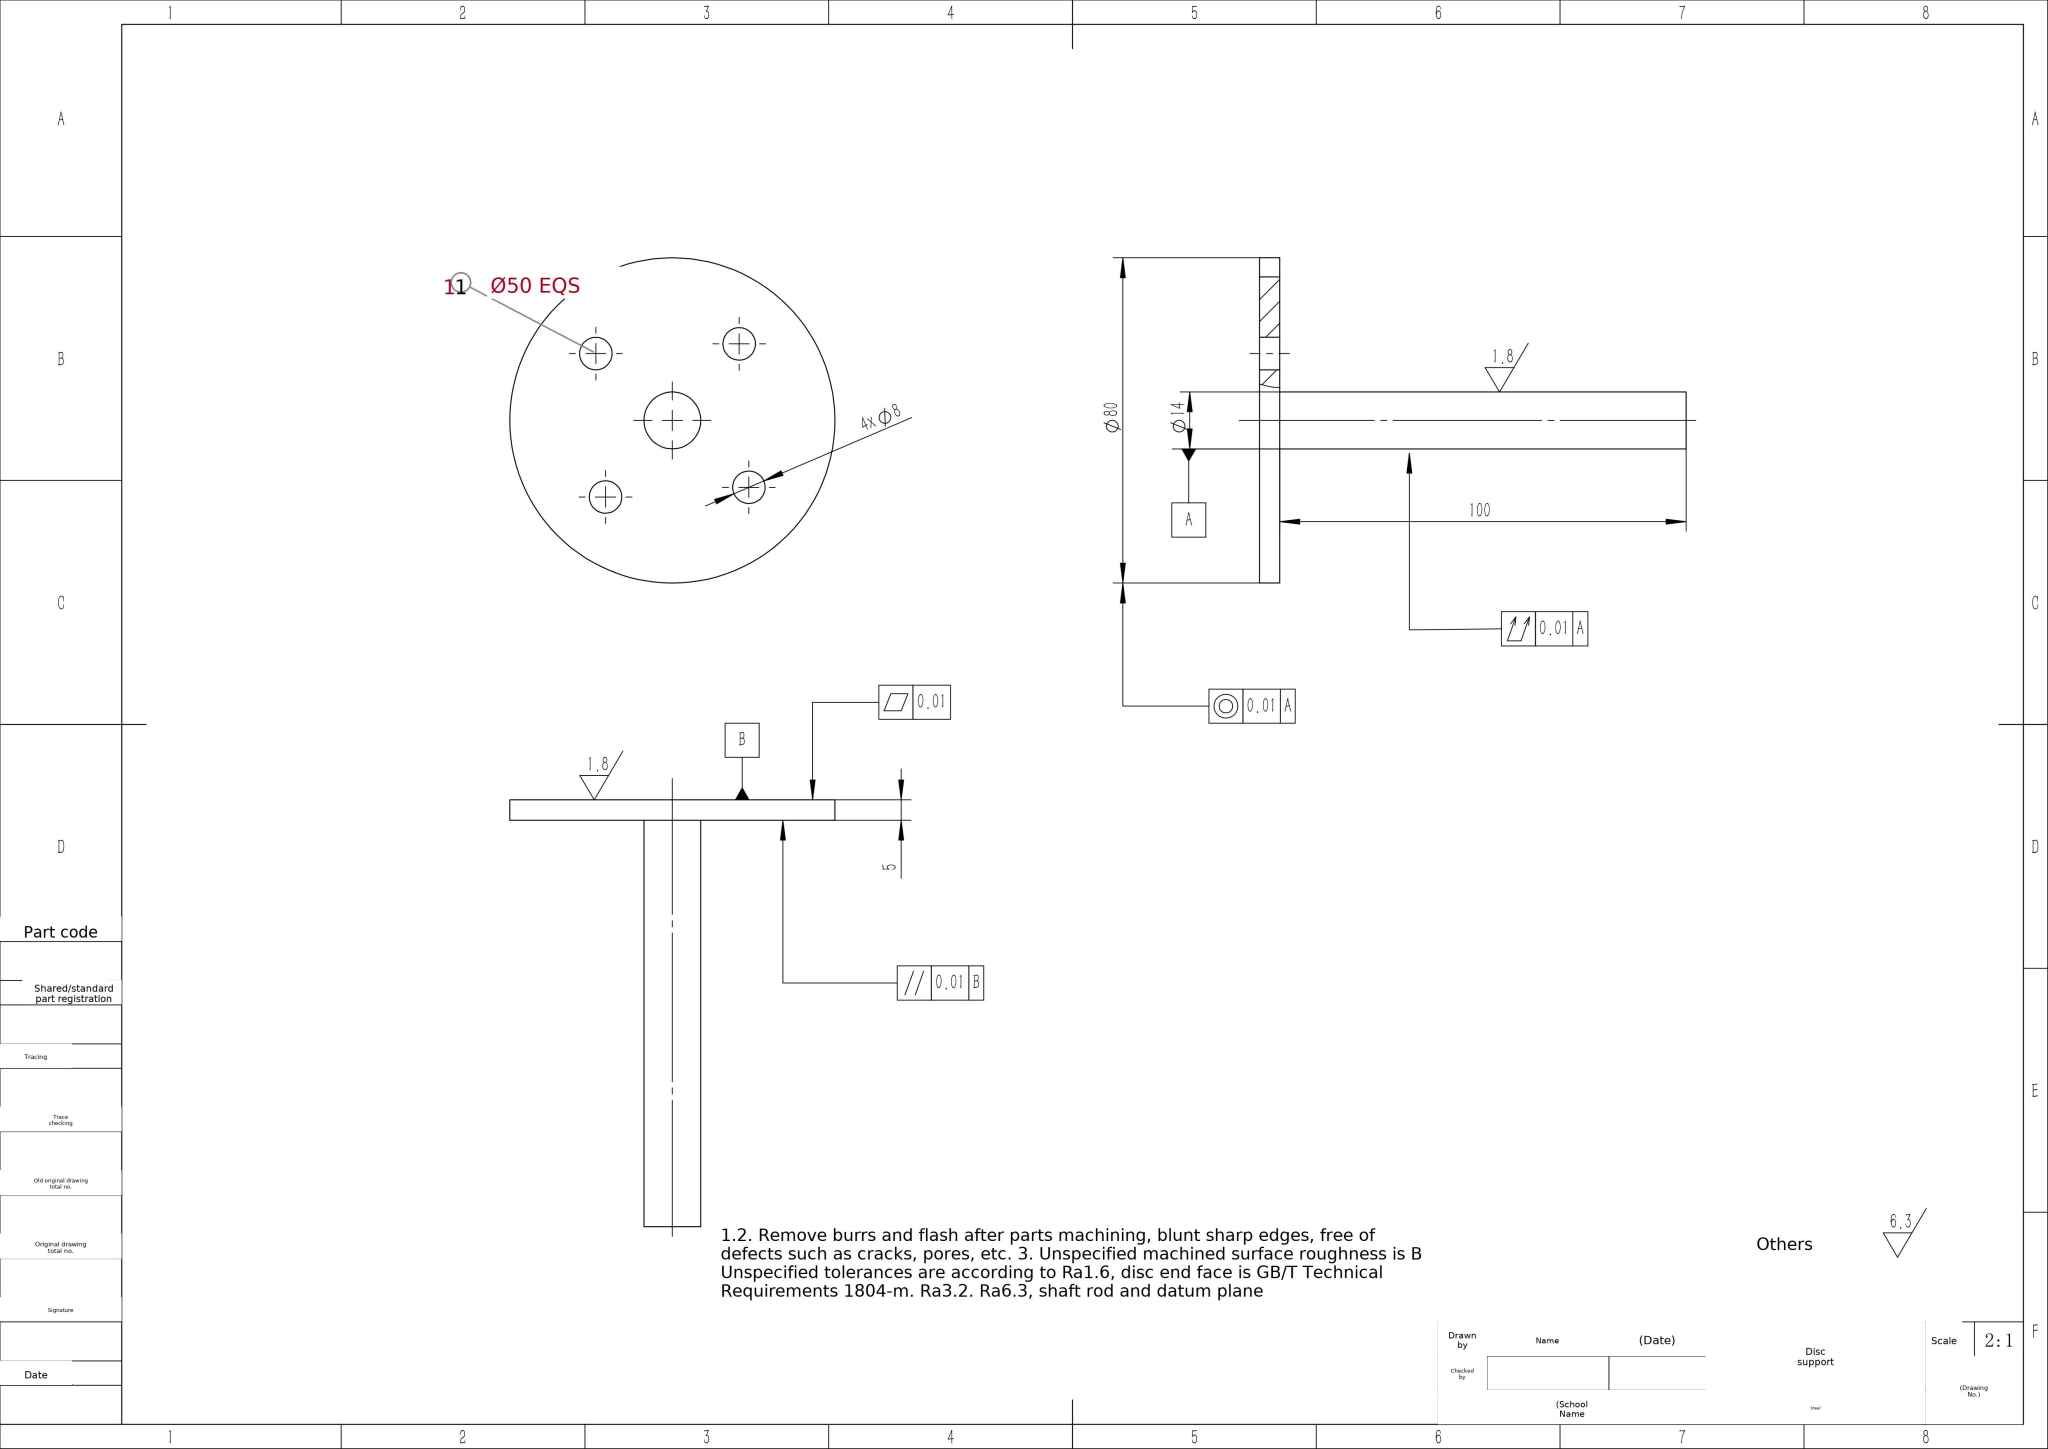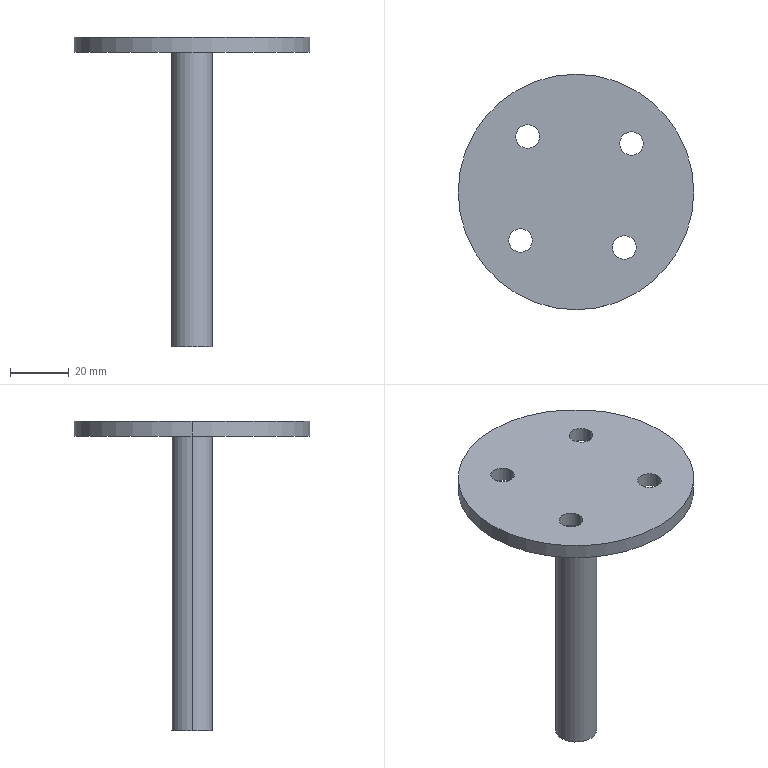Part | SolidWorks | mm | material Steel | 1 solid | 15 faces | box 80 x 80 x 105 mm | volume 39521 mm3 | cylinder 12 | plane 3 | commonest cylinder face diameters 8 x8 80 x2 14 x2
build123d program:
from build123d import *

# Parameters (mm, degrees)
SKETCH1_R           = 7
BOSS_EXTRUDE1_DEPTH = 100
SKETCH2_R           = 40
BOSS_EXTRUDE2_DEPTH = 5
SKETCH3_R           = 4
CUT_EXTRUDE1_DEPTH  = 5


with BuildPart() as part:
    # Sketch1 → Boss-Extrude1 (new body)
    with BuildSketch(Plane.XY):
        Circle(SKETCH1_R)
    extrude(amount=BOSS_EXTRUDE1_DEPTH)

    # Sketch2 → Boss-Extrude2 (add)
    with BuildSketch(Plane.XY.offset(100)):
        Circle(SKETCH2_R)
    extrude(amount=BOSS_EXTRUDE2_DEPTH)

    # Sketch3 → Cut-Extrude1 (cut)
    with BuildSketch(Plane.XY.offset(105)):
        with Locations((-16.444, 18.83)):
            Circle(SKETCH3_R)
        with Locations((18.83, 16.444)):
            Circle(SKETCH3_R)
        with Locations((16.444, -18.83)):
            Circle(SKETCH3_R)
        with Locations((-18.83, -16.444)):
            Circle(SKETCH3_R)
    extrude(amount=-CUT_EXTRUDE1_DEPTH, mode=Mode.SUBTRACT)


solid = part.part
STEP:
#1=CARTESIAN_POINT('',(14.83,16.444,100.));
#2=VERTEX_POINT('',#1);
#3=CARTESIAN_POINT('',(22.83,16.444,100.));
#4=VERTEX_POINT('',#3);
#5=CARTESIAN_POINT('',(18.83,16.444,100.));
#6=DIRECTION('',(0.,0.,1.));
#7=DIRECTION('',(1.,0.,0.));
#8=AXIS2_PLACEMENT_3D('',#5,#6,#7);
#9=CIRCLE('',#8,4.);
#10=EDGE_CURVE('',#2,#4,#9,.T.);
#11=ORIENTED_EDGE('',*,*,#10,.F.);
#12=CARTESIAN_POINT('',(14.83,16.444,105.));
#13=VERTEX_POINT('',#12);
#14=CARTESIAN_POINT('',(14.83,16.444,100.));
#15=DIRECTION('',(0.,0.,1.));
#16=VECTOR('',#15,1000.);
#17=LINE('',#14,#16);
#18=EDGE_CURVE('',#2,#13,#17,.T.);
#19=ORIENTED_EDGE('',*,*,#18,.T.);
#20=CARTESIAN_POINT('',(22.83,16.444,105.));
#21=VERTEX_POINT('',#20);
#22=CARTESIAN_POINT('',(18.83,16.444,105.));
#23=DIRECTION('',(0.,0.,1.));
#24=DIRECTION('',(1.,0.,0.));
#25=AXIS2_PLACEMENT_3D('',#22,#23,#24);
#26=CIRCLE('',#25,4.);
#27=EDGE_CURVE('',#13,#21,#26,.T.);
#28=ORIENTED_EDGE('',*,*,#27,.T.);
#29=CARTESIAN_POINT('',(22.83,16.444,100.));
#30=DIRECTION('',(0.,0.,1.));
#31=VECTOR('',#30,1000.);
#32=LINE('',#29,#31);
#33=EDGE_CURVE('',#4,#21,#32,.T.);
#34=ORIENTED_EDGE('',*,*,#33,.F.);
#35=EDGE_LOOP('',(#11,#19,#28,#34));
#36=FACE_OUTER_BOUND('',#35,.T.);
#37=CARTESIAN_POINT('',(18.83,16.444,100.));
#38=DIRECTION('',(0.,0.,1.));
#39=DIRECTION('',(1.,0.,0.));
#40=AXIS2_PLACEMENT_3D('',#37,#38,#39);
#41=CYLINDRICAL_SURFACE('',#40,4.);
#42=ADVANCED_FACE('',(#36),#41,.F.);
#43=CARTESIAN_POINT('',(12.444,-18.83,100.));
#44=VERTEX_POINT('',#43);
#45=CARTESIAN_POINT('',(20.444,-18.83,100.));
#46=VERTEX_POINT('',#45);
#47=CARTESIAN_POINT('',(16.444,-18.83,100.));
#48=DIRECTION('',(0.,0.,1.));
#49=DIRECTION('',(1.,0.,0.));
#50=AXIS2_PLACEMENT_3D('',#47,#48,#49);
#51=CIRCLE('',#50,4.);
#52=EDGE_CURVE('',#44,#46,#51,.T.);
#53=ORIENTED_EDGE('',*,*,#52,.F.);
#54=CARTESIAN_POINT('',(12.444,-18.83,105.));
#55=VERTEX_POINT('',#54);
#56=CARTESIAN_POINT('',(12.444,-18.83,100.));
#57=DIRECTION('',(0.,0.,1.));
#58=VECTOR('',#57,1000.);
#59=LINE('',#56,#58);
#60=EDGE_CURVE('',#44,#55,#59,.T.);
#61=ORIENTED_EDGE('',*,*,#60,.T.);
#62=CARTESIAN_POINT('',(20.444,-18.83,105.));
#63=VERTEX_POINT('',#62);
#64=CARTESIAN_POINT('',(16.444,-18.83,105.));
#65=DIRECTION('',(0.,0.,1.));
#66=DIRECTION('',(1.,0.,0.));
#67=AXIS2_PLACEMENT_3D('',#64,#65,#66);
#68=CIRCLE('',#67,4.);
#69=EDGE_CURVE('',#55,#63,#68,.T.);
#70=ORIENTED_EDGE('',*,*,#69,.T.);
#71=CARTESIAN_POINT('',(20.444,-18.83,100.));
#72=DIRECTION('',(0.,0.,1.));
#73=VECTOR('',#72,1000.);
#74=LINE('',#71,#73);
#75=EDGE_CURVE('',#46,#63,#74,.T.);
#76=ORIENTED_EDGE('',*,*,#75,.F.);
#77=EDGE_LOOP('',(#53,#61,#70,#76));
#78=FACE_OUTER_BOUND('',#77,.T.);
#79=CARTESIAN_POINT('',(16.444,-18.83,100.));
#80=DIRECTION('',(0.,0.,1.));
#81=DIRECTION('',(1.,0.,0.));
#82=AXIS2_PLACEMENT_3D('',#79,#80,#81);
#83=CYLINDRICAL_SURFACE('',#82,4.);
#84=ADVANCED_FACE('',(#78),#83,.F.);
#85=CARTESIAN_POINT('',(-22.83,-16.444,100.));
#86=VERTEX_POINT('',#85);
#87=CARTESIAN_POINT('',(-14.83,-16.444,100.));
#88=VERTEX_POINT('',#87);
#89=CARTESIAN_POINT('',(-18.83,-16.444,100.));
#90=DIRECTION('',(0.,0.,1.));
#91=DIRECTION('',(1.,0.,0.));
#92=AXIS2_PLACEMENT_3D('',#89,#90,#91);
#93=CIRCLE('',#92,4.);
#94=EDGE_CURVE('',#86,#88,#93,.T.);
#95=ORIENTED_EDGE('',*,*,#94,.F.);
#96=CARTESIAN_POINT('',(-22.83,-16.444,105.));
#97=VERTEX_POINT('',#96);
#98=CARTESIAN_POINT('',(-22.83,-16.444,100.));
#99=DIRECTION('',(0.,0.,1.));
#100=VECTOR('',#99,1000.);
#101=LINE('',#98,#100);
#102=EDGE_CURVE('',#86,#97,#101,.T.);
#103=ORIENTED_EDGE('',*,*,#102,.T.);
#104=CARTESIAN_POINT('',(-14.83,-16.444,105.));
#105=VERTEX_POINT('',#104);
#106=CARTESIAN_POINT('',(-18.83,-16.444,105.));
#107=DIRECTION('',(0.,0.,1.));
#108=DIRECTION('',(1.,0.,0.));
#109=AXIS2_PLACEMENT_3D('',#106,#107,#108);
#110=CIRCLE('',#109,4.);
#111=EDGE_CURVE('',#97,#105,#110,.T.);
#112=ORIENTED_EDGE('',*,*,#111,.T.);
#113=CARTESIAN_POINT('',(-14.83,-16.444,100.));
#114=DIRECTION('',(0.,0.,1.));
#115=VECTOR('',#114,1000.);
#116=LINE('',#113,#115);
#117=EDGE_CURVE('',#88,#105,#116,.T.);
#118=ORIENTED_EDGE('',*,*,#117,.F.);
#119=EDGE_LOOP('',(#95,#103,#112,#118));
#120=FACE_OUTER_BOUND('',#119,.T.);
#121=CARTESIAN_POINT('',(-18.83,-16.444,100.));
#122=DIRECTION('',(0.,0.,1.));
#123=DIRECTION('',(1.,0.,0.));
#124=AXIS2_PLACEMENT_3D('',#121,#122,#123);
#125=CYLINDRICAL_SURFACE('',#124,4.);
#126=ADVANCED_FACE('',(#120),#125,.F.);
#127=CARTESIAN_POINT('',(-20.444,18.83,100.));
#128=VERTEX_POINT('',#127);
#129=CARTESIAN_POINT('',(-12.444,18.83,100.));
#130=VERTEX_POINT('',#129);
#131=CARTESIAN_POINT('',(-16.444,18.83,100.));
#132=DIRECTION('',(0.,0.,1.));
#133=DIRECTION('',(1.,0.,0.));
#134=AXIS2_PLACEMENT_3D('',#131,#132,#133);
#135=CIRCLE('',#134,4.);
#136=EDGE_CURVE('',#128,#130,#135,.T.);
#137=ORIENTED_EDGE('',*,*,#136,.F.);
#138=CARTESIAN_POINT('',(-20.444,18.83,105.));
#139=VERTEX_POINT('',#138);
#140=CARTESIAN_POINT('',(-20.444,18.83,100.));
#141=DIRECTION('',(0.,0.,1.));
#142=VECTOR('',#141,1000.);
#143=LINE('',#140,#142);
#144=EDGE_CURVE('',#128,#139,#143,.T.);
#145=ORIENTED_EDGE('',*,*,#144,.T.);
#146=CARTESIAN_POINT('',(-12.444,18.83,105.));
#147=VERTEX_POINT('',#146);
#148=CARTESIAN_POINT('',(-16.444,18.83,105.));
#149=DIRECTION('',(0.,0.,1.));
#150=DIRECTION('',(1.,0.,0.));
#151=AXIS2_PLACEMENT_3D('',#148,#149,#150);
#152=CIRCLE('',#151,4.);
#153=EDGE_CURVE('',#139,#147,#152,.T.);
#154=ORIENTED_EDGE('',*,*,#153,.T.);
#155=CARTESIAN_POINT('',(-12.444,18.83,100.));
#156=DIRECTION('',(0.,0.,1.));
#157=VECTOR('',#156,1000.);
#158=LINE('',#155,#157);
#159=EDGE_CURVE('',#130,#147,#158,.T.);
#160=ORIENTED_EDGE('',*,*,#159,.F.);
#161=EDGE_LOOP('',(#137,#145,#154,#160));
#162=FACE_OUTER_BOUND('',#161,.T.);
#163=CARTESIAN_POINT('',(-16.444,18.83,100.));
#164=DIRECTION('',(0.,0.,1.));
#165=DIRECTION('',(1.,0.,0.));
#166=AXIS2_PLACEMENT_3D('',#163,#164,#165);
#167=CYLINDRICAL_SURFACE('',#166,4.);
#168=ADVANCED_FACE('',(#162),#167,.F.);
#169=CARTESIAN_POINT('',(40.,0.,105.));
#170=VERTEX_POINT('',#169);
#171=CARTESIAN_POINT('',(-40.,0.,105.));
#172=VERTEX_POINT('',#171);
#173=CARTESIAN_POINT('',(0.,0.,105.));
#174=DIRECTION('',(0.,0.,1.));
#175=DIRECTION('',(1.,0.,0.));
#176=AXIS2_PLACEMENT_3D('',#173,#174,#175);
#177=CIRCLE('',#176,40.);
#178=EDGE_CURVE('',#170,#172,#177,.T.);
#179=ORIENTED_EDGE('',*,*,#178,.F.);
#180=CARTESIAN_POINT('',(40.,0.,100.));
#181=VERTEX_POINT('',#180);
#182=CARTESIAN_POINT('',(40.,0.,105.));
#183=DIRECTION('',(0.,0.,-1.));
#184=VECTOR('',#183,1000.);
#185=LINE('',#182,#184);
#186=EDGE_CURVE('',#170,#181,#185,.T.);
#187=ORIENTED_EDGE('',*,*,#186,.T.);
#188=CARTESIAN_POINT('',(-40.,0.,100.));
#189=VERTEX_POINT('',#188);
#190=CARTESIAN_POINT('',(0.,0.,100.));
#191=DIRECTION('',(0.,0.,1.));
#192=DIRECTION('',(1.,0.,0.));
#193=AXIS2_PLACEMENT_3D('',#190,#191,#192);
#194=CIRCLE('',#193,40.);
#195=EDGE_CURVE('',#181,#189,#194,.T.);
#196=ORIENTED_EDGE('',*,*,#195,.T.);
#197=CARTESIAN_POINT('',(-40.,0.,105.));
#198=DIRECTION('',(0.,0.,-1.));
#199=VECTOR('',#198,1000.);
#200=LINE('',#197,#199);
#201=EDGE_CURVE('',#172,#189,#200,.T.);
#202=ORIENTED_EDGE('',*,*,#201,.F.);
#203=EDGE_LOOP('',(#179,#187,#196,#202));
#204=FACE_OUTER_BOUND('',#203,.T.);
#205=CARTESIAN_POINT('',(0.,0.,105.));
#206=DIRECTION('',(0.,0.,-1.));
#207=DIRECTION('',(-1.,0.,0.));
#208=AXIS2_PLACEMENT_3D('',#205,#206,#207);
#209=CYLINDRICAL_SURFACE('',#208,40.);
#210=ADVANCED_FACE('',(#204),#209,.T.);
#211=CARTESIAN_POINT('',(7.,0.,100.));
#212=VERTEX_POINT('',#211);
#213=CARTESIAN_POINT('',(-7.,0.,100.));
#214=VERTEX_POINT('',#213);
#215=CARTESIAN_POINT('',(0.,0.,100.));
#216=DIRECTION('',(0.,0.,1.));
#217=DIRECTION('',(1.,0.,0.));
#218=AXIS2_PLACEMENT_3D('',#215,#216,#217);
#219=CIRCLE('',#218,7.);
#220=EDGE_CURVE('',#212,#214,#219,.T.);
#221=ORIENTED_EDGE('',*,*,#220,.F.);
#222=CARTESIAN_POINT('',(7.,0.,0.));
#223=VERTEX_POINT('',#222);
#224=CARTESIAN_POINT('',(7.,0.,100.));
#225=DIRECTION('',(0.,0.,-1.));
#226=VECTOR('',#225,1000.);
#227=LINE('',#224,#226);
#228=EDGE_CURVE('',#212,#223,#227,.T.);
#229=ORIENTED_EDGE('',*,*,#228,.T.);
#230=CARTESIAN_POINT('',(-7.,0.,0.));
#231=VERTEX_POINT('',#230);
#232=CARTESIAN_POINT('',(0.,0.,0.));
#233=DIRECTION('',(0.,0.,1.));
#234=DIRECTION('',(1.,0.,0.));
#235=AXIS2_PLACEMENT_3D('',#232,#233,#234);
#236=CIRCLE('',#235,7.);
#237=EDGE_CURVE('',#223,#231,#236,.T.);
#238=ORIENTED_EDGE('',*,*,#237,.T.);
#239=CARTESIAN_POINT('',(-7.,0.,100.));
#240=DIRECTION('',(0.,0.,-1.));
#241=VECTOR('',#240,1000.);
#242=LINE('',#239,#241);
#243=EDGE_CURVE('',#214,#231,#242,.T.);
#244=ORIENTED_EDGE('',*,*,#243,.F.);
#245=EDGE_LOOP('',(#221,#229,#238,#244));
#246=FACE_OUTER_BOUND('',#245,.T.);
#247=CARTESIAN_POINT('',(0.,0.,100.));
#248=DIRECTION('',(0.,0.,-1.));
#249=DIRECTION('',(-1.,0.,0.));
#250=AXIS2_PLACEMENT_3D('',#247,#248,#249);
#251=CYLINDRICAL_SURFACE('',#250,7.);
#252=ADVANCED_FACE('',(#246),#251,.T.);
#253=ORIENTED_EDGE('',*,*,#228,.F.);
#254=CARTESIAN_POINT('',(0.,0.,100.));
#255=DIRECTION('',(0.,0.,1.));
#256=DIRECTION('',(1.,0.,0.));
#257=AXIS2_PLACEMENT_3D('',#254,#255,#256);
#258=CIRCLE('',#257,7.);
#259=EDGE_CURVE('',#214,#212,#258,.T.);
#260=ORIENTED_EDGE('',*,*,#259,.F.);
#261=ORIENTED_EDGE('',*,*,#243,.T.);
#262=CARTESIAN_POINT('',(0.,0.,0.));
#263=DIRECTION('',(0.,0.,1.));
#264=DIRECTION('',(1.,0.,0.));
#265=AXIS2_PLACEMENT_3D('',#262,#263,#264);
#266=CIRCLE('',#265,7.);
#267=EDGE_CURVE('',#231,#223,#266,.T.);
#268=ORIENTED_EDGE('',*,*,#267,.T.);
#269=EDGE_LOOP('',(#253,#260,#261,#268));
#270=FACE_OUTER_BOUND('',#269,.T.);
#271=CARTESIAN_POINT('',(0.,0.,100.));
#272=DIRECTION('',(0.,0.,-1.));
#273=DIRECTION('',(-1.,0.,0.));
#274=AXIS2_PLACEMENT_3D('',#271,#272,#273);
#275=CYLINDRICAL_SURFACE('',#274,7.);
#276=ADVANCED_FACE('',(#270),#275,.T.);
#277=ORIENTED_EDGE('',*,*,#267,.F.);
#278=ORIENTED_EDGE('',*,*,#237,.F.);
#279=EDGE_LOOP('',(#277,#278));
#280=FACE_OUTER_BOUND('',#279,.T.);
#281=CARTESIAN_POINT('',(0.,0.,0.));
#282=DIRECTION('',(0.,0.,1.));
#283=DIRECTION('',(1.,0.,0.));
#284=AXIS2_PLACEMENT_3D('',#281,#282,#283);
#285=PLANE('',#284);
#286=ADVANCED_FACE('',(#280),#285,.F.);
#287=ORIENTED_EDGE('',*,*,#186,.F.);
#288=CARTESIAN_POINT('',(0.,0.,105.));
#289=DIRECTION('',(0.,0.,1.));
#290=DIRECTION('',(1.,0.,0.));
#291=AXIS2_PLACEMENT_3D('',#288,#289,#290);
#292=CIRCLE('',#291,40.);
#293=EDGE_CURVE('',#172,#170,#292,.T.);
#294=ORIENTED_EDGE('',*,*,#293,.F.);
#295=ORIENTED_EDGE('',*,*,#201,.T.);
#296=CARTESIAN_POINT('',(0.,0.,100.));
#297=DIRECTION('',(0.,0.,1.));
#298=DIRECTION('',(1.,0.,0.));
#299=AXIS2_PLACEMENT_3D('',#296,#297,#298);
#300=CIRCLE('',#299,40.);
#301=EDGE_CURVE('',#189,#181,#300,.T.);
#302=ORIENTED_EDGE('',*,*,#301,.T.);
#303=EDGE_LOOP('',(#287,#294,#295,#302));
#304=FACE_OUTER_BOUND('',#303,.T.);
#305=CARTESIAN_POINT('',(0.,0.,105.));
#306=DIRECTION('',(0.,0.,-1.));
#307=DIRECTION('',(-1.,0.,0.));
#308=AXIS2_PLACEMENT_3D('',#305,#306,#307);
#309=CYLINDRICAL_SURFACE('',#308,40.);
#310=ADVANCED_FACE('',(#304),#309,.T.);
#311=CARTESIAN_POINT('',(18.83,16.444,105.));
#312=DIRECTION('',(0.,0.,1.));
#313=DIRECTION('',(1.,0.,0.));
#314=AXIS2_PLACEMENT_3D('',#311,#312,#313);
#315=CIRCLE('',#314,4.);
#316=EDGE_CURVE('',#21,#13,#315,.T.);
#317=ORIENTED_EDGE('',*,*,#316,.F.);
#318=ORIENTED_EDGE('',*,*,#27,.F.);
#319=EDGE_LOOP('',(#317,#318));
#320=FACE_BOUND('',#319,.T.);
#321=CARTESIAN_POINT('',(16.444,-18.83,105.));
#322=DIRECTION('',(0.,0.,1.));
#323=DIRECTION('',(1.,0.,0.));
#324=AXIS2_PLACEMENT_3D('',#321,#322,#323);
#325=CIRCLE('',#324,4.);
#326=EDGE_CURVE('',#63,#55,#325,.T.);
#327=ORIENTED_EDGE('',*,*,#326,.F.);
#328=ORIENTED_EDGE('',*,*,#69,.F.);
#329=EDGE_LOOP('',(#327,#328));
#330=FACE_BOUND('',#329,.T.);
#331=CARTESIAN_POINT('',(-18.83,-16.444,105.));
#332=DIRECTION('',(0.,0.,1.));
#333=DIRECTION('',(1.,0.,0.));
#334=AXIS2_PLACEMENT_3D('',#331,#332,#333);
#335=CIRCLE('',#334,4.);
#336=EDGE_CURVE('',#105,#97,#335,.T.);
#337=ORIENTED_EDGE('',*,*,#336,.F.);
#338=ORIENTED_EDGE('',*,*,#111,.F.);
#339=EDGE_LOOP('',(#337,#338));
#340=FACE_BOUND('',#339,.T.);
#341=CARTESIAN_POINT('',(-16.444,18.83,105.));
#342=DIRECTION('',(0.,0.,1.));
#343=DIRECTION('',(1.,0.,0.));
#344=AXIS2_PLACEMENT_3D('',#341,#342,#343);
#345=CIRCLE('',#344,4.);
#346=EDGE_CURVE('',#147,#139,#345,.T.);
#347=ORIENTED_EDGE('',*,*,#346,.F.);
#348=ORIENTED_EDGE('',*,*,#153,.F.);
#349=EDGE_LOOP('',(#347,#348));
#350=FACE_BOUND('',#349,.T.);
#351=ORIENTED_EDGE('',*,*,#293,.T.);
#352=ORIENTED_EDGE('',*,*,#178,.T.);
#353=EDGE_LOOP('',(#351,#352));
#354=FACE_OUTER_BOUND('',#353,.T.);
#355=CARTESIAN_POINT('',(0.,0.,105.));
#356=DIRECTION('',(0.,0.,1.));
#357=DIRECTION('',(1.,0.,0.));
#358=AXIS2_PLACEMENT_3D('',#355,#356,#357);
#359=PLANE('',#358);
#360=ADVANCED_FACE('',(#320,#330,#340,#350,#354),#359,.T.);
#361=CARTESIAN_POINT('',(18.83,16.444,100.));
#362=DIRECTION('',(0.,0.,1.));
#363=DIRECTION('',(1.,0.,0.));
#364=AXIS2_PLACEMENT_3D('',#361,#362,#363);
#365=CIRCLE('',#364,4.);
#366=EDGE_CURVE('',#4,#2,#365,.T.);
#367=ORIENTED_EDGE('',*,*,#366,.T.);
#368=ORIENTED_EDGE('',*,*,#10,.T.);
#369=EDGE_LOOP('',(#367,#368));
#370=FACE_BOUND('',#369,.T.);
#371=CARTESIAN_POINT('',(16.444,-18.83,100.));
#372=DIRECTION('',(0.,0.,1.));
#373=DIRECTION('',(1.,0.,0.));
#374=AXIS2_PLACEMENT_3D('',#371,#372,#373);
#375=CIRCLE('',#374,4.);
#376=EDGE_CURVE('',#46,#44,#375,.T.);
#377=ORIENTED_EDGE('',*,*,#376,.T.);
#378=ORIENTED_EDGE('',*,*,#52,.T.);
#379=EDGE_LOOP('',(#377,#378));
#380=FACE_BOUND('',#379,.T.);
#381=CARTESIAN_POINT('',(-18.83,-16.444,100.));
#382=DIRECTION('',(0.,0.,1.));
#383=DIRECTION('',(1.,0.,0.));
#384=AXIS2_PLACEMENT_3D('',#381,#382,#383);
#385=CIRCLE('',#384,4.);
#386=EDGE_CURVE('',#88,#86,#385,.T.);
#387=ORIENTED_EDGE('',*,*,#386,.T.);
#388=ORIENTED_EDGE('',*,*,#94,.T.);
#389=EDGE_LOOP('',(#387,#388));
#390=FACE_BOUND('',#389,.T.);
#391=CARTESIAN_POINT('',(-16.444,18.83,100.));
#392=DIRECTION('',(0.,0.,1.));
#393=DIRECTION('',(1.,0.,0.));
#394=AXIS2_PLACEMENT_3D('',#391,#392,#393);
#395=CIRCLE('',#394,4.);
#396=EDGE_CURVE('',#130,#128,#395,.T.);
#397=ORIENTED_EDGE('',*,*,#396,.T.);
#398=ORIENTED_EDGE('',*,*,#136,.T.);
#399=EDGE_LOOP('',(#397,#398));
#400=FACE_BOUND('',#399,.T.);
#401=ORIENTED_EDGE('',*,*,#259,.T.);
#402=ORIENTED_EDGE('',*,*,#220,.T.);
#403=EDGE_LOOP('',(#401,#402));
#404=FACE_BOUND('',#403,.T.);
#405=ORIENTED_EDGE('',*,*,#301,.F.);
#406=ORIENTED_EDGE('',*,*,#195,.F.);
#407=EDGE_LOOP('',(#405,#406));
#408=FACE_OUTER_BOUND('',#407,.T.);
#409=CARTESIAN_POINT('',(0.,0.,100.));
#410=DIRECTION('',(0.,0.,1.));
#411=DIRECTION('',(1.,0.,0.));
#412=AXIS2_PLACEMENT_3D('',#409,#410,#411);
#413=PLANE('',#412);
#414=ADVANCED_FACE('',(#370,#380,#390,#400,#404,#408),#413,.F.);
#415=ORIENTED_EDGE('',*,*,#144,.F.);
#416=ORIENTED_EDGE('',*,*,#396,.F.);
#417=ORIENTED_EDGE('',*,*,#159,.T.);
#418=ORIENTED_EDGE('',*,*,#346,.T.);
#419=EDGE_LOOP('',(#415,#416,#417,#418));
#420=FACE_OUTER_BOUND('',#419,.T.);
#421=CARTESIAN_POINT('',(-16.444,18.83,100.));
#422=DIRECTION('',(0.,0.,1.));
#423=DIRECTION('',(1.,0.,0.));
#424=AXIS2_PLACEMENT_3D('',#421,#422,#423);
#425=CYLINDRICAL_SURFACE('',#424,4.);
#426=ADVANCED_FACE('',(#420),#425,.F.);
#427=ORIENTED_EDGE('',*,*,#102,.F.);
#428=ORIENTED_EDGE('',*,*,#386,.F.);
#429=ORIENTED_EDGE('',*,*,#117,.T.);
#430=ORIENTED_EDGE('',*,*,#336,.T.);
#431=EDGE_LOOP('',(#427,#428,#429,#430));
#432=FACE_OUTER_BOUND('',#431,.T.);
#433=CARTESIAN_POINT('',(-18.83,-16.444,100.));
#434=DIRECTION('',(0.,0.,1.));
#435=DIRECTION('',(1.,0.,0.));
#436=AXIS2_PLACEMENT_3D('',#433,#434,#435);
#437=CYLINDRICAL_SURFACE('',#436,4.);
#438=ADVANCED_FACE('',(#432),#437,.F.);
#439=ORIENTED_EDGE('',*,*,#60,.F.);
#440=ORIENTED_EDGE('',*,*,#376,.F.);
#441=ORIENTED_EDGE('',*,*,#75,.T.);
#442=ORIENTED_EDGE('',*,*,#326,.T.);
#443=EDGE_LOOP('',(#439,#440,#441,#442));
#444=FACE_OUTER_BOUND('',#443,.T.);
#445=CARTESIAN_POINT('',(16.444,-18.83,100.));
#446=DIRECTION('',(0.,0.,1.));
#447=DIRECTION('',(1.,0.,0.));
#448=AXIS2_PLACEMENT_3D('',#445,#446,#447);
#449=CYLINDRICAL_SURFACE('',#448,4.);
#450=ADVANCED_FACE('',(#444),#449,.F.);
#451=ORIENTED_EDGE('',*,*,#18,.F.);
#452=ORIENTED_EDGE('',*,*,#366,.F.);
#453=ORIENTED_EDGE('',*,*,#33,.T.);
#454=ORIENTED_EDGE('',*,*,#316,.T.);
#455=EDGE_LOOP('',(#451,#452,#453,#454));
#456=FACE_OUTER_BOUND('',#455,.T.);
#457=CARTESIAN_POINT('',(18.83,16.444,100.));
#458=DIRECTION('',(0.,0.,1.));
#459=DIRECTION('',(1.,0.,0.));
#460=AXIS2_PLACEMENT_3D('',#457,#458,#459);
#461=CYLINDRICAL_SURFACE('',#460,4.);
#462=ADVANCED_FACE('',(#456),#461,.F.);
#463=CLOSED_SHELL('',(#42,#84,#126,#168,#210,#252,#276,#286,#310,#360,#414,#426,#438,#450,#462));
#464=MANIFOLD_SOLID_BREP('',#463);
#465=CARTESIAN_POINT('',(0.,0.,0.));
#466=DIRECTION('',(0.,0.,1.));
#467=DIRECTION('',(1.,0.,0.));
#468=AXIS2_PLACEMENT_3D('',#465,#466,#467);
#469=(LENGTH_UNIT()NAMED_UNIT(*)SI_UNIT(.MILLI.,.METRE.));
#470=UNCERTAINTY_MEASURE_WITH_UNIT(LENGTH_MEASURE(0.00001),#469,'','');
#471=(NAMED_UNIT(*)PLANE_ANGLE_UNIT()SI_UNIT($,.RADIAN.));
#472=(NAMED_UNIT(*)SI_UNIT($,.STERADIAN.)SOLID_ANGLE_UNIT());
#473=(GEOMETRIC_REPRESENTATION_CONTEXT(3)GLOBAL_UNCERTAINTY_ASSIGNED_CONTEXT((#470))GLOBAL_UNIT_ASSIGNED_CONTEXT((#469,#471,#472))REPRESENTATION_CONTEXT('',''));
#474=ADVANCED_BREP_SHAPE_REPRESENTATION('',(#464,#468),#473);